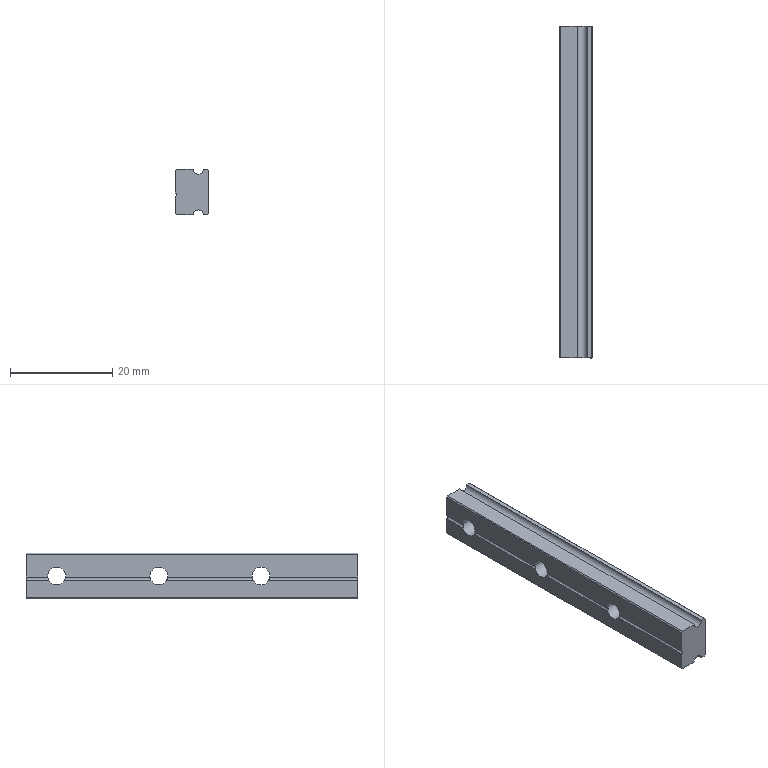Component | SolidWorks | XMGN9C-70GuideRail--D-2 | 1 solid | 35 faces | volume 3202 mm3 | cylinder 19 | plane 16 | commonest cylinder face diameters 6 x6 3.5 x6 0.6 x4 2 x3